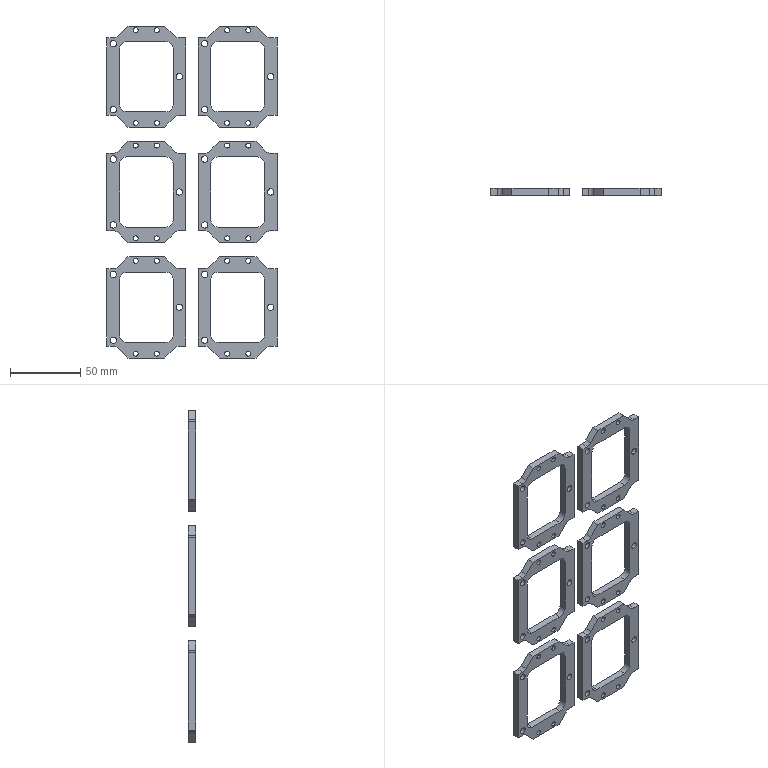CAM job | Mastercam | mm | 5 operations | part box 121 x 5 x 236
1. Contour (Ramp) | 3 - 3 平铣刀
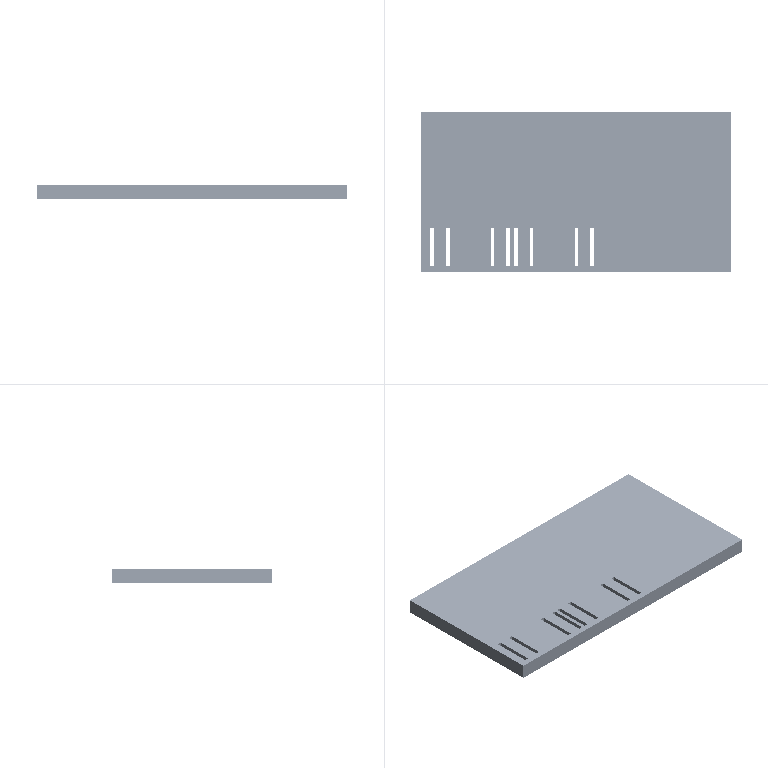2. Drill/Counterbore | 5 - 4 倒角刀
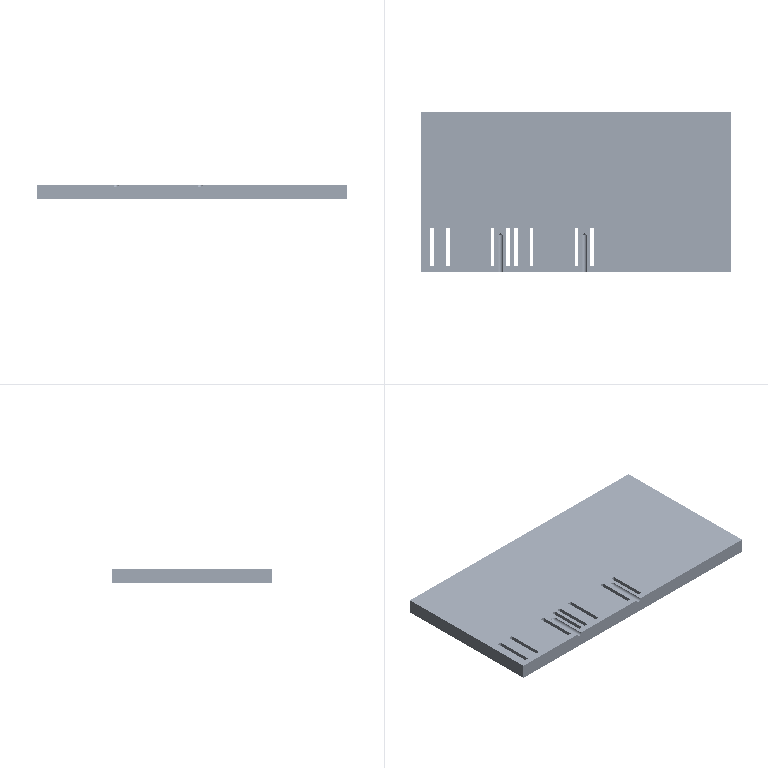3. Contour (2D chamfer) | 5 - 4 倒角刀
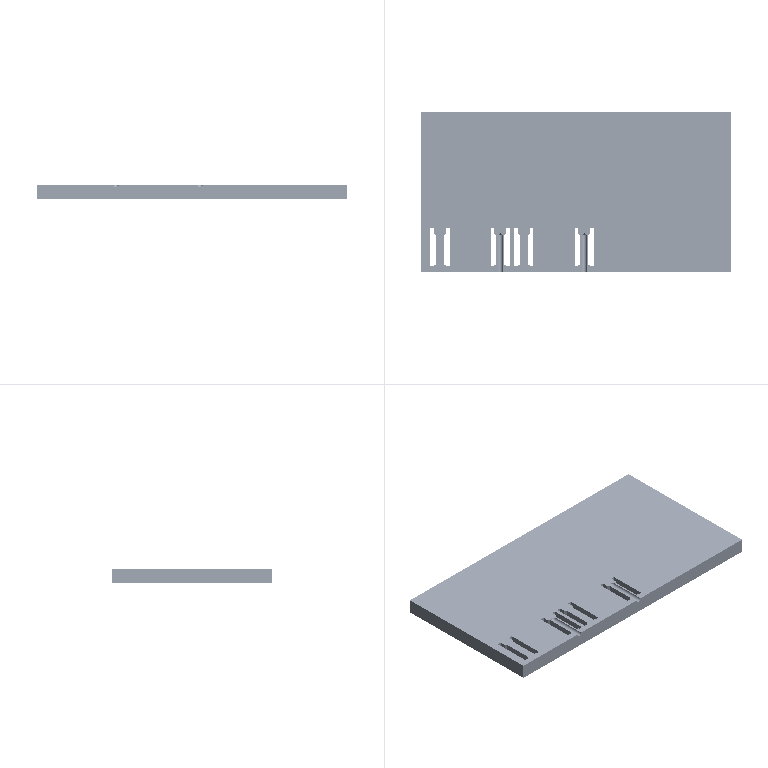4. Contour (Ramp) | 2 - 2 平铣刀
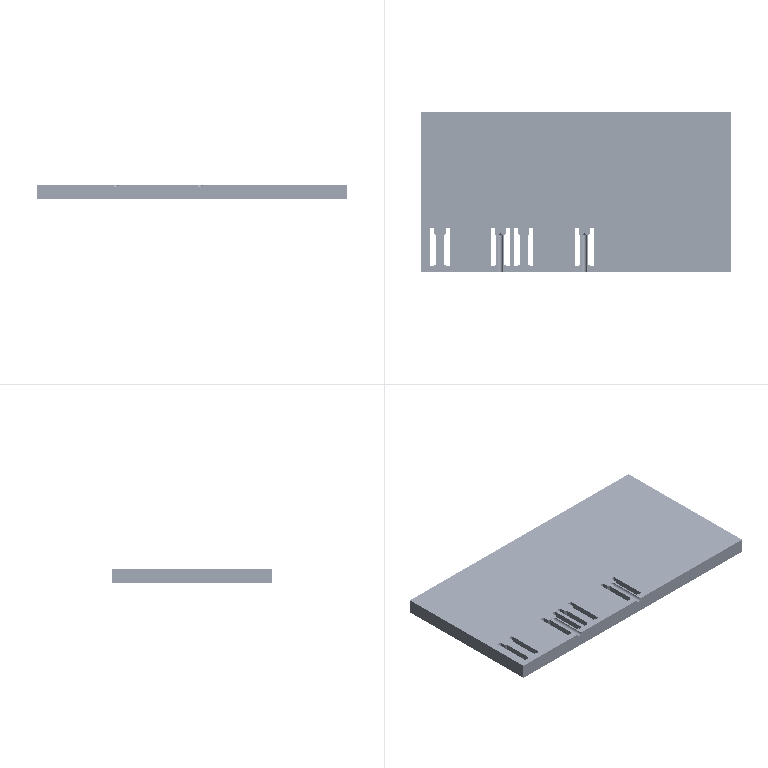5. Contour (2D chamfer) | 5 - 4 倒角刀